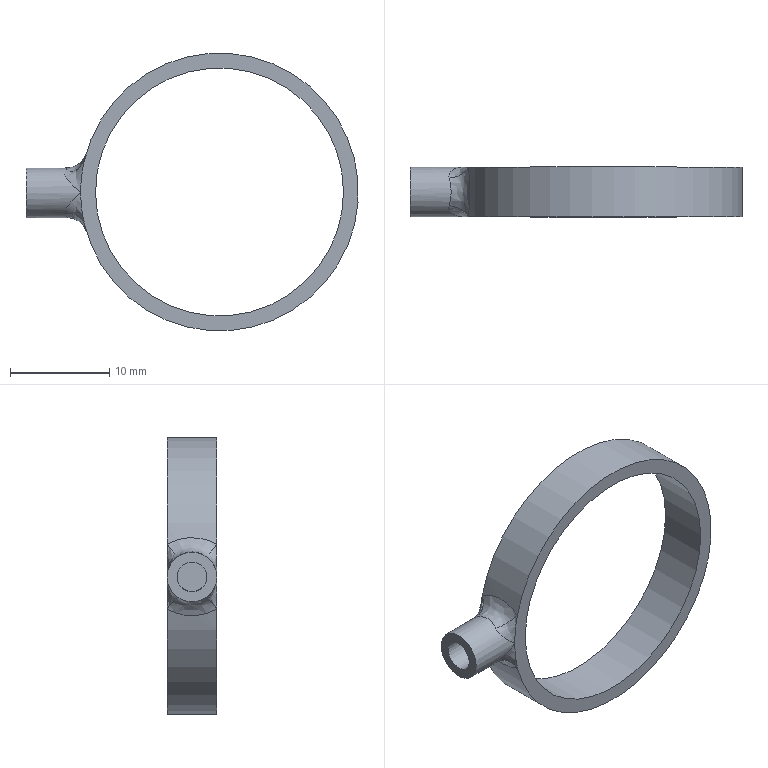Component | NX | LINK_5_RING | 1 solid | 14 faces | volume 693 mm3 | spline 6 | cylinder 4 | plane 4 | commonest cylinder face diameters 28 x1 25 x1 5 x1 3 x1